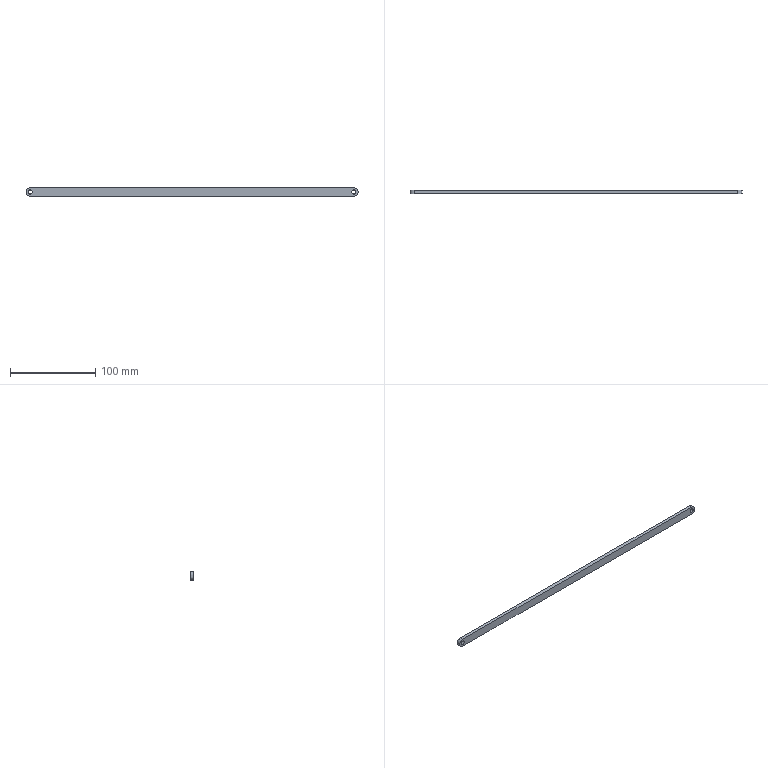Component | NX | LINK | 1 solid | 8 faces | box 390 x 4 x 10 mm | volume 15357 mm3 | cylinder 4 | plane 4 | commonest cylinder face diameters 10 x2 5 x2
STEP:
#1=CARTESIAN_POINT('',(0.,0.,0.));
#2=DIRECTION('',(0.,0.,1.));
#3=DIRECTION('',(1.,0.,0.));
#4=AXIS2_PLACEMENT_3D('',#1,#2,#3);
#5=CARTESIAN_POINT('',(447.686,493.538,-37.155));
#6=VERTEX_POINT('',#5);
#7=CARTESIAN_POINT('',(447.686,493.538,-47.155));
#8=VERTEX_POINT('',#7);
#9=CARTESIAN_POINT('',(447.686,493.538,-42.155));
#10=DIRECTION('',(0.,1.,0.));
#11=DIRECTION('',(-1.,0.,0.));
#12=AXIS2_PLACEMENT_3D('',#9,#10,#11);
#13=CIRCLE('',#12,5.);
#14=CARTESIAN_POINT('',(447.686,497.538,-42.155));
#15=DIRECTION('',(0.,-1.,0.));
#16=DIRECTION('',(0.,0.,1.));
#17=AXIS2_PLACEMENT_3D('',#14,#15,#16);
#18=CYLINDRICAL_SURFACE('',#17,5.);
#19=CARTESIAN_POINT('',(7.854,4.));
#20=DIRECTION('',(-1.,0.));
#21=VECTOR('',#20,1.);
#22=LINE('',#19,#21);
#23=(GEOMETRIC_REPRESENTATION_CONTEXT(2)PARAMETRIC_REPRESENTATION_CONTEXT()REPRESENTATION_CONTEXT('',''));
#24=DEFINITIONAL_REPRESENTATION('',(#22),#23);
#25=PCURVE('',#18,#24);
#26=CARTESIAN_POINT('',(447.686,493.538,-42.155));
#27=DIRECTION('',(0.,1.,0.));
#28=DIRECTION('',(0.,0.,-1.));
#29=AXIS2_PLACEMENT_3D('',#26,#27,#28);
#30=PLANE('',#29);
#31=CARTESIAN_POINT('',(0.,0.));
#32=DIRECTION('',(0.,1.));
#33=AXIS2_PLACEMENT_2D('',#31,#32);
#34=CIRCLE('',#33,5.);
#35=(GEOMETRIC_REPRESENTATION_CONTEXT(2)PARAMETRIC_REPRESENTATION_CONTEXT()REPRESENTATION_CONTEXT('',''));
#36=DEFINITIONAL_REPRESENTATION('',(#34),#35);
#37=PCURVE('',#30,#36);
#38=SURFACE_CURVE('',#13,(#25,#37),.PCURVE_S1.);
#39=EDGE_CURVE('',#6,#8,#38,.T.);
#40=ORIENTED_EDGE('',*,*,#39,.T.);
#41=CARTESIAN_POINT('',(447.686,497.538,-47.155));
#42=VERTEX_POINT('',#41);
#43=CARTESIAN_POINT('',(447.686,497.538,-47.155));
#44=DIRECTION('',(0.,-1.,0.));
#45=VECTOR('',#44,1.);
#46=LINE('',#43,#45);
#47=CARTESIAN_POINT('',(3.142,0.));
#48=DIRECTION('',(0.,1.));
#49=VECTOR('',#48,1.);
#50=LINE('',#47,#49);
#51=(GEOMETRIC_REPRESENTATION_CONTEXT(2)PARAMETRIC_REPRESENTATION_CONTEXT()REPRESENTATION_CONTEXT('',''));
#52=DEFINITIONAL_REPRESENTATION('',(#50),#51);
#53=PCURVE('',#18,#52);
#54=CARTESIAN_POINT('',(447.686,497.538,-47.155));
#55=DIRECTION('',(0.,0.,1.));
#56=DIRECTION('',(0.,1.,0.));
#57=AXIS2_PLACEMENT_3D('',#54,#55,#56);
#58=PLANE('',#57);
#59=CARTESIAN_POINT('',(0.,0.));
#60=DIRECTION('',(-1.,0.));
#61=VECTOR('',#60,1.);
#62=LINE('',#59,#61);
#63=(GEOMETRIC_REPRESENTATION_CONTEXT(2)PARAMETRIC_REPRESENTATION_CONTEXT()REPRESENTATION_CONTEXT('',''));
#64=DEFINITIONAL_REPRESENTATION('',(#62),#63);
#65=PCURVE('',#58,#64);
#66=SURFACE_CURVE('',#46,(#53,#65),.PCURVE_S1.);
#67=EDGE_CURVE('',#42,#8,#66,.T.);
#68=ORIENTED_EDGE('',*,*,#67,.F.);
#69=CARTESIAN_POINT('',(447.686,497.538,-37.155));
#70=VERTEX_POINT('',#69);
#71=CARTESIAN_POINT('',(447.686,497.538,-42.155));
#72=DIRECTION('',(0.,1.,0.));
#73=DIRECTION('',(-1.,0.,0.));
#74=AXIS2_PLACEMENT_3D('',#71,#72,#73);
#75=CIRCLE('',#74,5.);
#76=CARTESIAN_POINT('',(7.854,0.));
#77=DIRECTION('',(-1.,0.));
#78=VECTOR('',#77,1.);
#79=LINE('',#76,#78);
#80=(GEOMETRIC_REPRESENTATION_CONTEXT(2)PARAMETRIC_REPRESENTATION_CONTEXT()REPRESENTATION_CONTEXT('',''));
#81=DEFINITIONAL_REPRESENTATION('',(#79),#80);
#82=PCURVE('',#18,#81);
#83=CARTESIAN_POINT('',(447.686,497.538,-42.155));
#84=DIRECTION('',(0.,1.,0.));
#85=DIRECTION('',(0.,0.,-1.));
#86=AXIS2_PLACEMENT_3D('',#83,#84,#85);
#87=PLANE('',#86);
#88=CARTESIAN_POINT('',(0.,0.));
#89=DIRECTION('',(0.,1.));
#90=AXIS2_PLACEMENT_2D('',#88,#89);
#91=CIRCLE('',#90,5.);
#92=(GEOMETRIC_REPRESENTATION_CONTEXT(2)PARAMETRIC_REPRESENTATION_CONTEXT()REPRESENTATION_CONTEXT('',''));
#93=DEFINITIONAL_REPRESENTATION('',(#91),#92);
#94=PCURVE('',#87,#93);
#95=SURFACE_CURVE('',#75,(#82,#94),.PCURVE_S1.);
#96=EDGE_CURVE('',#70,#42,#95,.T.);
#97=ORIENTED_EDGE('',*,*,#96,.F.);
#98=CARTESIAN_POINT('',(447.686,497.538,-37.155));
#99=DIRECTION('',(0.,-1.,0.));
#100=VECTOR('',#99,1.);
#101=LINE('',#98,#100);
#102=CARTESIAN_POINT('',(6.283,0.));
#103=DIRECTION('',(0.,1.));
#104=VECTOR('',#103,1.);
#105=LINE('',#102,#104);
#106=(GEOMETRIC_REPRESENTATION_CONTEXT(2)PARAMETRIC_REPRESENTATION_CONTEXT()REPRESENTATION_CONTEXT('',''));
#107=DEFINITIONAL_REPRESENTATION('',(#105),#106);
#108=PCURVE('',#18,#107);
#109=CARTESIAN_POINT('',(67.686,497.538,-37.155));
#110=DIRECTION('',(0.,0.,-1.));
#111=DIRECTION('',(0.,-1.,0.));
#112=AXIS2_PLACEMENT_3D('',#109,#110,#111);
#113=PLANE('',#112);
#114=CARTESIAN_POINT('',(0.,-380.));
#115=DIRECTION('',(1.,0.));
#116=VECTOR('',#115,1.);
#117=LINE('',#114,#116);
#118=(GEOMETRIC_REPRESENTATION_CONTEXT(2)PARAMETRIC_REPRESENTATION_CONTEXT()REPRESENTATION_CONTEXT('',''));
#119=DEFINITIONAL_REPRESENTATION('',(#117),#118);
#120=PCURVE('',#113,#119);
#121=SURFACE_CURVE('',#101,(#108,#120),.PCURVE_S1.);
#122=EDGE_CURVE('',#70,#6,#121,.T.);
#123=ORIENTED_EDGE('',*,*,#122,.T.);
#124=EDGE_LOOP('',(#40,#68,#97,#123));
#125=FACE_BOUND('',#124,.T.);
#126=ADVANCED_FACE('',(#125),#18,.T.);
#127=CARTESIAN_POINT('',(67.686,493.538,-47.155));
#128=VERTEX_POINT('',#127);
#129=CARTESIAN_POINT('',(447.686,493.538,-47.155));
#130=DIRECTION('',(-1.,0.,0.));
#131=VECTOR('',#130,1.);
#132=LINE('',#129,#131);
#133=CARTESIAN_POINT('',(-4.,0.));
#134=DIRECTION('',(0.,1.));
#135=VECTOR('',#134,1.);
#136=LINE('',#133,#135);
#137=(GEOMETRIC_REPRESENTATION_CONTEXT(2)PARAMETRIC_REPRESENTATION_CONTEXT()REPRESENTATION_CONTEXT('',''));
#138=DEFINITIONAL_REPRESENTATION('',(#136),#137);
#139=PCURVE('',#58,#138);
#140=CARTESIAN_POINT('',(5.,0.));
#141=DIRECTION('',(0.,1.));
#142=VECTOR('',#141,1.);
#143=LINE('',#140,#142);
#144=(GEOMETRIC_REPRESENTATION_CONTEXT(2)PARAMETRIC_REPRESENTATION_CONTEXT()REPRESENTATION_CONTEXT('',''));
#145=DEFINITIONAL_REPRESENTATION('',(#143),#144);
#146=PCURVE('',#30,#145);
#147=SURFACE_CURVE('',#132,(#139,#146),.PCURVE_S1.);
#148=EDGE_CURVE('',#8,#128,#147,.T.);
#149=ORIENTED_EDGE('',*,*,#148,.T.);
#150=CARTESIAN_POINT('',(67.686,497.538,-47.155));
#151=VERTEX_POINT('',#150);
#152=CARTESIAN_POINT('',(67.686,497.538,-47.155));
#153=DIRECTION('',(0.,-1.,0.));
#154=VECTOR('',#153,1.);
#155=LINE('',#152,#154);
#156=CARTESIAN_POINT('',(0.,380.));
#157=DIRECTION('',(-1.,0.));
#158=VECTOR('',#157,1.);
#159=LINE('',#156,#158);
#160=(GEOMETRIC_REPRESENTATION_CONTEXT(2)PARAMETRIC_REPRESENTATION_CONTEXT()REPRESENTATION_CONTEXT('',''));
#161=DEFINITIONAL_REPRESENTATION('',(#159),#160);
#162=PCURVE('',#58,#161);
#163=CARTESIAN_POINT('',(67.686,497.538,-42.155));
#164=DIRECTION('',(0.,-1.,0.));
#165=DIRECTION('',(0.,0.,1.));
#166=AXIS2_PLACEMENT_3D('',#163,#164,#165);
#167=CYLINDRICAL_SURFACE('',#166,5.);
#168=CARTESIAN_POINT('',(3.142,0.));
#169=DIRECTION('',(0.,1.));
#170=VECTOR('',#169,1.);
#171=LINE('',#168,#170);
#172=(GEOMETRIC_REPRESENTATION_CONTEXT(2)PARAMETRIC_REPRESENTATION_CONTEXT()REPRESENTATION_CONTEXT('',''));
#173=DEFINITIONAL_REPRESENTATION('',(#171),#172);
#174=PCURVE('',#167,#173);
#175=SURFACE_CURVE('',#155,(#162,#174),.PCURVE_S1.);
#176=EDGE_CURVE('',#151,#128,#175,.T.);
#177=ORIENTED_EDGE('',*,*,#176,.F.);
#178=CARTESIAN_POINT('',(447.686,497.538,-47.155));
#179=DIRECTION('',(-1.,0.,0.));
#180=VECTOR('',#179,1.);
#181=LINE('',#178,#180);
#182=CARTESIAN_POINT('',(0.,0.));
#183=DIRECTION('',(0.,1.));
#184=VECTOR('',#183,1.);
#185=LINE('',#182,#184);
#186=(GEOMETRIC_REPRESENTATION_CONTEXT(2)PARAMETRIC_REPRESENTATION_CONTEXT()REPRESENTATION_CONTEXT('',''));
#187=DEFINITIONAL_REPRESENTATION('',(#185),#186);
#188=PCURVE('',#58,#187);
#189=CARTESIAN_POINT('',(5.,0.));
#190=DIRECTION('',(0.,1.));
#191=VECTOR('',#190,1.);
#192=LINE('',#189,#191);
#193=(GEOMETRIC_REPRESENTATION_CONTEXT(2)PARAMETRIC_REPRESENTATION_CONTEXT()REPRESENTATION_CONTEXT('',''));
#194=DEFINITIONAL_REPRESENTATION('',(#192),#193);
#195=PCURVE('',#87,#194);
#196=SURFACE_CURVE('',#181,(#188,#195),.PCURVE_S1.);
#197=EDGE_CURVE('',#42,#151,#196,.T.);
#198=ORIENTED_EDGE('',*,*,#197,.F.);
#199=ORIENTED_EDGE('',*,*,#67,.T.);
#200=EDGE_LOOP('',(#149,#177,#198,#199));
#201=FACE_BOUND('',#200,.T.);
#202=ADVANCED_FACE('',(#201),#58,.F.);
#203=CARTESIAN_POINT('',(67.686,493.538,-37.155));
#204=VERTEX_POINT('',#203);
#205=CARTESIAN_POINT('',(67.686,493.538,-42.155));
#206=DIRECTION('',(0.,1.,0.));
#207=DIRECTION('',(-1.,0.,0.));
#208=AXIS2_PLACEMENT_3D('',#205,#206,#207);
#209=CIRCLE('',#208,5.);
#210=CARTESIAN_POINT('',(7.854,4.));
#211=DIRECTION('',(-1.,0.));
#212=VECTOR('',#211,1.);
#213=LINE('',#210,#212);
#214=(GEOMETRIC_REPRESENTATION_CONTEXT(2)PARAMETRIC_REPRESENTATION_CONTEXT()REPRESENTATION_CONTEXT('',''));
#215=DEFINITIONAL_REPRESENTATION('',(#213),#214);
#216=PCURVE('',#167,#215);
#217=CARTESIAN_POINT('',(0.,380.));
#218=DIRECTION('',(0.,1.));
#219=AXIS2_PLACEMENT_2D('',#217,#218);
#220=CIRCLE('',#219,5.);
#221=(GEOMETRIC_REPRESENTATION_CONTEXT(2)PARAMETRIC_REPRESENTATION_CONTEXT()REPRESENTATION_CONTEXT('',''));
#222=DEFINITIONAL_REPRESENTATION('',(#220),#221);
#223=PCURVE('',#30,#222);
#224=SURFACE_CURVE('',#209,(#216,#223),.PCURVE_S1.);
#225=EDGE_CURVE('',#128,#204,#224,.T.);
#226=ORIENTED_EDGE('',*,*,#225,.T.);
#227=CARTESIAN_POINT('',(67.686,497.538,-37.155));
#228=VERTEX_POINT('',#227);
#229=CARTESIAN_POINT('',(67.686,497.538,-37.155));
#230=DIRECTION('',(0.,-1.,0.));
#231=VECTOR('',#230,1.);
#232=LINE('',#229,#231);
#233=CARTESIAN_POINT('',(0.,0.));
#234=DIRECTION('',(0.,1.));
#235=VECTOR('',#234,1.);
#236=LINE('',#233,#235);
#237=(GEOMETRIC_REPRESENTATION_CONTEXT(2)PARAMETRIC_REPRESENTATION_CONTEXT()REPRESENTATION_CONTEXT('',''));
#238=DEFINITIONAL_REPRESENTATION('',(#236),#237);
#239=PCURVE('',#167,#238);
#240=CARTESIAN_POINT('',(0.,0.));
#241=DIRECTION('',(1.,0.));
#242=VECTOR('',#241,1.);
#243=LINE('',#240,#242);
#244=(GEOMETRIC_REPRESENTATION_CONTEXT(2)PARAMETRIC_REPRESENTATION_CONTEXT()REPRESENTATION_CONTEXT('',''));
#245=DEFINITIONAL_REPRESENTATION('',(#243),#244);
#246=PCURVE('',#113,#245);
#247=SURFACE_CURVE('',#232,(#239,#246),.PCURVE_S1.);
#248=EDGE_CURVE('',#228,#204,#247,.T.);
#249=ORIENTED_EDGE('',*,*,#248,.F.);
#250=CARTESIAN_POINT('',(67.686,497.538,-42.155));
#251=DIRECTION('',(0.,1.,0.));
#252=DIRECTION('',(-1.,0.,0.));
#253=AXIS2_PLACEMENT_3D('',#250,#251,#252);
#254=CIRCLE('',#253,5.);
#255=CARTESIAN_POINT('',(7.854,0.));
#256=DIRECTION('',(-1.,0.));
#257=VECTOR('',#256,1.);
#258=LINE('',#255,#257);
#259=(GEOMETRIC_REPRESENTATION_CONTEXT(2)PARAMETRIC_REPRESENTATION_CONTEXT()REPRESENTATION_CONTEXT('',''));
#260=DEFINITIONAL_REPRESENTATION('',(#258),#259);
#261=PCURVE('',#167,#260);
#262=CARTESIAN_POINT('',(0.,380.));
#263=DIRECTION('',(0.,1.));
#264=AXIS2_PLACEMENT_2D('',#262,#263);
#265=CIRCLE('',#264,5.);
#266=(GEOMETRIC_REPRESENTATION_CONTEXT(2)PARAMETRIC_REPRESENTATION_CONTEXT()REPRESENTATION_CONTEXT('',''));
#267=DEFINITIONAL_REPRESENTATION('',(#265),#266);
#268=PCURVE('',#87,#267);
#269=SURFACE_CURVE('',#254,(#261,#268),.PCURVE_S1.);
#270=EDGE_CURVE('',#151,#228,#269,.T.);
#271=ORIENTED_EDGE('',*,*,#270,.F.);
#272=ORIENTED_EDGE('',*,*,#176,.T.);
#273=EDGE_LOOP('',(#226,#249,#271,#272));
#274=FACE_BOUND('',#273,.T.);
#275=ADVANCED_FACE('',(#274),#167,.T.);
#276=CARTESIAN_POINT('',(445.186,497.538,-42.155));
#277=VERTEX_POINT('',#276);
#278=CARTESIAN_POINT('',(447.686,497.538,-42.155));
#279=DIRECTION('',(0.,1.,0.));
#280=DIRECTION('',(-1.,0.,0.));
#281=AXIS2_PLACEMENT_3D('',#278,#279,#280);
#282=CIRCLE('',#281,2.5);
#283=CARTESIAN_POINT('',(447.686,497.538,-42.155));
#284=DIRECTION('',(0.,-1.,0.));
#285=DIRECTION('',(0.,0.,1.));
#286=AXIS2_PLACEMENT_3D('',#283,#284,#285);
#287=CYLINDRICAL_SURFACE('',#286,2.5);
#288=CARTESIAN_POINT('',(7.854,0.));
#289=DIRECTION('',(-1.,0.));
#290=VECTOR('',#289,1.);
#291=LINE('',#288,#290);
#292=(GEOMETRIC_REPRESENTATION_CONTEXT(2)PARAMETRIC_REPRESENTATION_CONTEXT()REPRESENTATION_CONTEXT('',''));
#293=DEFINITIONAL_REPRESENTATION('',(#291),#292);
#294=PCURVE('',#287,#293);
#295=CARTESIAN_POINT('',(0.,0.));
#296=DIRECTION('',(0.,1.));
#297=AXIS2_PLACEMENT_2D('',#295,#296);
#298=CIRCLE('',#297,2.5);
#299=(GEOMETRIC_REPRESENTATION_CONTEXT(2)PARAMETRIC_REPRESENTATION_CONTEXT()REPRESENTATION_CONTEXT('',''));
#300=DEFINITIONAL_REPRESENTATION('',(#298),#299);
#301=PCURVE('',#87,#300);
#302=SURFACE_CURVE('',#282,(#294,#301),.PCURVE_S1.);
#303=EDGE_CURVE('',#277,#277,#302,.T.);
#304=ORIENTED_EDGE('',*,*,#303,.F.);
#305=CARTESIAN_POINT('',(445.186,493.538,-42.155));
#306=VERTEX_POINT('',#305);
#307=CARTESIAN_POINT('',(445.186,497.538,-42.155));
#308=CARTESIAN_POINT('',(445.186,493.538,-42.155));
#309=B_SPLINE_CURVE_WITH_KNOTS('',1,(#307,#308),.UNSPECIFIED.,.F.,.F.,(2,2),(0.,4.),.PIECEWISE_BEZIER_KNOTS.);
#310=CARTESIAN_POINT('',(7.854,0.));
#311=DIRECTION('',(0.,1.));
#312=VECTOR('',#311,1.);
#313=LINE('',#310,#312);
#314=(GEOMETRIC_REPRESENTATION_CONTEXT(2)PARAMETRIC_REPRESENTATION_CONTEXT()REPRESENTATION_CONTEXT('',''));
#315=DEFINITIONAL_REPRESENTATION('',(#313),#314);
#316=PCURVE('',#287,#315);
#317=CARTESIAN_POINT('',(1.571,0.));
#318=DIRECTION('',(0.,1.));
#319=VECTOR('',#318,1.);
#320=LINE('',#317,#319);
#321=(GEOMETRIC_REPRESENTATION_CONTEXT(2)PARAMETRIC_REPRESENTATION_CONTEXT()REPRESENTATION_CONTEXT('',''));
#322=DEFINITIONAL_REPRESENTATION('',(#320),#321);
#323=PCURVE('',#287,#322);
#324=SEAM_CURVE('',#309,(#316,#323),.PCURVE_S1.);
#325=EDGE_CURVE('',#277,#306,#324,.T.);
#326=ORIENTED_EDGE('',*,*,#325,.T.);
#327=CARTESIAN_POINT('',(447.686,493.538,-42.155));
#328=DIRECTION('',(0.,1.,0.));
#329=DIRECTION('',(-1.,0.,0.));
#330=AXIS2_PLACEMENT_3D('',#327,#328,#329);
#331=CIRCLE('',#330,2.5);
#332=CARTESIAN_POINT('',(7.854,4.));
#333=DIRECTION('',(-1.,0.));
#334=VECTOR('',#333,1.);
#335=LINE('',#332,#334);
#336=(GEOMETRIC_REPRESENTATION_CONTEXT(2)PARAMETRIC_REPRESENTATION_CONTEXT()REPRESENTATION_CONTEXT('',''));
#337=DEFINITIONAL_REPRESENTATION('',(#335),#336);
#338=PCURVE('',#287,#337);
#339=CARTESIAN_POINT('',(0.,0.));
#340=DIRECTION('',(0.,1.));
#341=AXIS2_PLACEMENT_2D('',#339,#340);
#342=CIRCLE('',#341,2.5);
#343=(GEOMETRIC_REPRESENTATION_CONTEXT(2)PARAMETRIC_REPRESENTATION_CONTEXT()REPRESENTATION_CONTEXT('',''));
#344=DEFINITIONAL_REPRESENTATION('',(#342),#343);
#345=PCURVE('',#30,#344);
#346=SURFACE_CURVE('',#331,(#338,#345),.PCURVE_S1.);
#347=EDGE_CURVE('',#306,#306,#346,.T.);
#348=ORIENTED_EDGE('',*,*,#347,.T.);
#349=ORIENTED_EDGE('',*,*,#325,.F.);
#350=EDGE_LOOP('',(#304,#326,#348,#349));
#351=FACE_BOUND('',#350,.F.);
#352=ADVANCED_FACE('',(#351),#287,.F.);
#353=CARTESIAN_POINT('',(67.686,493.538,-37.155));
#354=DIRECTION('',(1.,0.,0.));
#355=VECTOR('',#354,1.);
#356=LINE('',#353,#355);
#357=CARTESIAN_POINT('',(4.,0.));
#358=DIRECTION('',(0.,-1.));
#359=VECTOR('',#358,1.);
#360=LINE('',#357,#359);
#361=(GEOMETRIC_REPRESENTATION_CONTEXT(2)PARAMETRIC_REPRESENTATION_CONTEXT()REPRESENTATION_CONTEXT('',''));
#362=DEFINITIONAL_REPRESENTATION('',(#360),#361);
#363=PCURVE('',#113,#362);
#364=CARTESIAN_POINT('',(-5.,380.));
#365=DIRECTION('',(0.,-1.));
#366=VECTOR('',#365,1.);
#367=LINE('',#364,#366);
#368=(GEOMETRIC_REPRESENTATION_CONTEXT(2)PARAMETRIC_REPRESENTATION_CONTEXT()REPRESENTATION_CONTEXT('',''));
#369=DEFINITIONAL_REPRESENTATION('',(#367),#368);
#370=PCURVE('',#30,#369);
#371=SURFACE_CURVE('',#356,(#363,#370),.PCURVE_S1.);
#372=EDGE_CURVE('',#204,#6,#371,.T.);
#373=ORIENTED_EDGE('',*,*,#372,.T.);
#374=ORIENTED_EDGE('',*,*,#122,.F.);
#375=CARTESIAN_POINT('',(67.686,497.538,-37.155));
#376=DIRECTION('',(1.,0.,0.));
#377=VECTOR('',#376,1.);
#378=LINE('',#375,#377);
#379=CARTESIAN_POINT('',(0.,0.));
#380=DIRECTION('',(0.,-1.));
#381=VECTOR('',#380,1.);
#382=LINE('',#379,#381);
#383=(GEOMETRIC_REPRESENTATION_CONTEXT(2)PARAMETRIC_REPRESENTATION_CONTEXT()REPRESENTATION_CONTEXT('',''));
#384=DEFINITIONAL_REPRESENTATION('',(#382),#383);
#385=PCURVE('',#113,#384);
#386=CARTESIAN_POINT('',(-5.,380.));
#387=DIRECTION('',(0.,-1.));
#388=VECTOR('',#387,1.);
#389=LINE('',#386,#388);
#390=(GEOMETRIC_REPRESENTATION_CONTEXT(2)PARAMETRIC_REPRESENTATION_CONTEXT()REPRESENTATION_CONTEXT('',''));
#391=DEFINITIONAL_REPRESENTATION('',(#389),#390);
#392=PCURVE('',#87,#391);
#393=SURFACE_CURVE('',#378,(#385,#392),.PCURVE_S1.);
#394=EDGE_CURVE('',#228,#70,#393,.T.);
#395=ORIENTED_EDGE('',*,*,#394,.F.);
#396=ORIENTED_EDGE('',*,*,#248,.T.);
#397=EDGE_LOOP('',(#373,#374,#395,#396));
#398=FACE_BOUND('',#397,.T.);
#399=ADVANCED_FACE('',(#398),#113,.F.);
#400=CARTESIAN_POINT('',(65.186,497.538,-42.155));
#401=VERTEX_POINT('',#400);
#402=CARTESIAN_POINT('',(67.686,497.538,-42.155));
#403=DIRECTION('',(0.,1.,0.));
#404=DIRECTION('',(-1.,0.,0.));
#405=AXIS2_PLACEMENT_3D('',#402,#403,#404);
#406=CIRCLE('',#405,2.5);
#407=CARTESIAN_POINT('',(67.686,497.538,-42.155));
#408=DIRECTION('',(0.,-1.,0.));
#409=DIRECTION('',(0.,0.,1.));
#410=AXIS2_PLACEMENT_3D('',#407,#408,#409);
#411=CYLINDRICAL_SURFACE('',#410,2.5);
#412=CARTESIAN_POINT('',(7.854,0.));
#413=DIRECTION('',(-1.,0.));
#414=VECTOR('',#413,1.);
#415=LINE('',#412,#414);
#416=(GEOMETRIC_REPRESENTATION_CONTEXT(2)PARAMETRIC_REPRESENTATION_CONTEXT()REPRESENTATION_CONTEXT('',''));
#417=DEFINITIONAL_REPRESENTATION('',(#415),#416);
#418=PCURVE('',#411,#417);
#419=CARTESIAN_POINT('',(0.,380.));
#420=DIRECTION('',(0.,1.));
#421=AXIS2_PLACEMENT_2D('',#419,#420);
#422=CIRCLE('',#421,2.5);
#423=(GEOMETRIC_REPRESENTATION_CONTEXT(2)PARAMETRIC_REPRESENTATION_CONTEXT()REPRESENTATION_CONTEXT('',''));
#424=DEFINITIONAL_REPRESENTATION('',(#422),#423);
#425=PCURVE('',#87,#424);
#426=SURFACE_CURVE('',#406,(#418,#425),.PCURVE_S1.);
#427=EDGE_CURVE('',#401,#401,#426,.T.);
#428=ORIENTED_EDGE('',*,*,#427,.F.);
#429=CARTESIAN_POINT('',(65.186,493.538,-42.155));
#430=VERTEX_POINT('',#429);
#431=CARTESIAN_POINT('',(65.186,497.538,-42.155));
#432=CARTESIAN_POINT('',(65.186,493.538,-42.155));
#433=B_SPLINE_CURVE_WITH_KNOTS('',1,(#431,#432),.UNSPECIFIED.,.F.,.F.,(2,2),(0.,4.),.PIECEWISE_BEZIER_KNOTS.);
#434=CARTESIAN_POINT('',(7.854,0.));
#435=DIRECTION('',(0.,1.));
#436=VECTOR('',#435,1.);
#437=LINE('',#434,#436);
#438=(GEOMETRIC_REPRESENTATION_CONTEXT(2)PARAMETRIC_REPRESENTATION_CONTEXT()REPRESENTATION_CONTEXT('',''));
#439=DEFINITIONAL_REPRESENTATION('',(#437),#438);
#440=PCURVE('',#411,#439);
#441=CARTESIAN_POINT('',(1.571,0.));
#442=DIRECTION('',(0.,1.));
#443=VECTOR('',#442,1.);
#444=LINE('',#441,#443);
#445=(GEOMETRIC_REPRESENTATION_CONTEXT(2)PARAMETRIC_REPRESENTATION_CONTEXT()REPRESENTATION_CONTEXT('',''));
#446=DEFINITIONAL_REPRESENTATION('',(#444),#445);
#447=PCURVE('',#411,#446);
#448=SEAM_CURVE('',#433,(#440,#447),.PCURVE_S1.);
#449=EDGE_CURVE('',#401,#430,#448,.T.);
#450=ORIENTED_EDGE('',*,*,#449,.T.);
#451=CARTESIAN_POINT('',(67.686,493.538,-42.155));
#452=DIRECTION('',(0.,1.,0.));
#453=DIRECTION('',(-1.,0.,0.));
#454=AXIS2_PLACEMENT_3D('',#451,#452,#453);
#455=CIRCLE('',#454,2.5);
#456=CARTESIAN_POINT('',(7.854,4.));
#457=DIRECTION('',(-1.,0.));
#458=VECTOR('',#457,1.);
#459=LINE('',#456,#458);
#460=(GEOMETRIC_REPRESENTATION_CONTEXT(2)PARAMETRIC_REPRESENTATION_CONTEXT()REPRESENTATION_CONTEXT('',''));
#461=DEFINITIONAL_REPRESENTATION('',(#459),#460);
#462=PCURVE('',#411,#461);
#463=CARTESIAN_POINT('',(0.,380.));
#464=DIRECTION('',(0.,1.));
#465=AXIS2_PLACEMENT_2D('',#463,#464);
#466=CIRCLE('',#465,2.5);
#467=(GEOMETRIC_REPRESENTATION_CONTEXT(2)PARAMETRIC_REPRESENTATION_CONTEXT()REPRESENTATION_CONTEXT('',''));
#468=DEFINITIONAL_REPRESENTATION('',(#466),#467);
#469=PCURVE('',#30,#468);
#470=SURFACE_CURVE('',#455,(#462,#469),.PCURVE_S1.);
#471=EDGE_CURVE('',#430,#430,#470,.T.);
#472=ORIENTED_EDGE('',*,*,#471,.T.);
#473=ORIENTED_EDGE('',*,*,#449,.F.);
#474=EDGE_LOOP('',(#428,#450,#472,#473));
#475=FACE_BOUND('',#474,.F.);
#476=ADVANCED_FACE('',(#475),#411,.F.);
#477=ORIENTED_EDGE('',*,*,#96,.T.);
#478=ORIENTED_EDGE('',*,*,#197,.T.);
#479=ORIENTED_EDGE('',*,*,#270,.T.);
#480=ORIENTED_EDGE('',*,*,#394,.T.);
#481=EDGE_LOOP('',(#477,#478,#479,#480));
#482=FACE_BOUND('',#481,.T.);
#483=ORIENTED_EDGE('',*,*,#303,.F.);
#484=EDGE_LOOP('',(#483));
#485=FACE_BOUND('',#484,.T.);
#486=ORIENTED_EDGE('',*,*,#427,.F.);
#487=EDGE_LOOP('',(#486));
#488=FACE_BOUND('',#487,.T.);
#489=ADVANCED_FACE('',(#482,#485,#488),#87,.T.);
#490=ORIENTED_EDGE('',*,*,#39,.F.);
#491=ORIENTED_EDGE('',*,*,#372,.F.);
#492=ORIENTED_EDGE('',*,*,#225,.F.);
#493=ORIENTED_EDGE('',*,*,#148,.F.);
#494=EDGE_LOOP('',(#490,#491,#492,#493));
#495=FACE_BOUND('',#494,.T.);
#496=ORIENTED_EDGE('',*,*,#347,.T.);
#497=EDGE_LOOP('',(#496));
#498=FACE_BOUND('',#497,.T.);
#499=ORIENTED_EDGE('',*,*,#471,.T.);
#500=EDGE_LOOP('',(#499));
#501=FACE_BOUND('',#500,.T.);
#502=ADVANCED_FACE('',(#495,#498,#501),#30,.F.);
#503=CLOSED_SHELL('',(#126,#202,#275,#352,#399,#476,#489,#502));
#504=MANIFOLD_SOLID_BREP('',#503);
#505=(LENGTH_UNIT()NAMED_UNIT(*)SI_UNIT(.MILLI.,.METRE.));
#506=UNCERTAINTY_MEASURE_WITH_UNIT(LENGTH_MEASURE(0.000002),#505,'','');
#507=(NAMED_UNIT(*)PLANE_ANGLE_UNIT()SI_UNIT($,.RADIAN.));
#508=(NAMED_UNIT(*)SI_UNIT($,.STERADIAN.)SOLID_ANGLE_UNIT());
#509=(GEOMETRIC_REPRESENTATION_CONTEXT(3)GLOBAL_UNCERTAINTY_ASSIGNED_CONTEXT((#506))GLOBAL_UNIT_ASSIGNED_CONTEXT((#505,#507,#508))REPRESENTATION_CONTEXT('',''));
#510=ADVANCED_BREP_SHAPE_REPRESENTATION('',(#4,#504),#509);